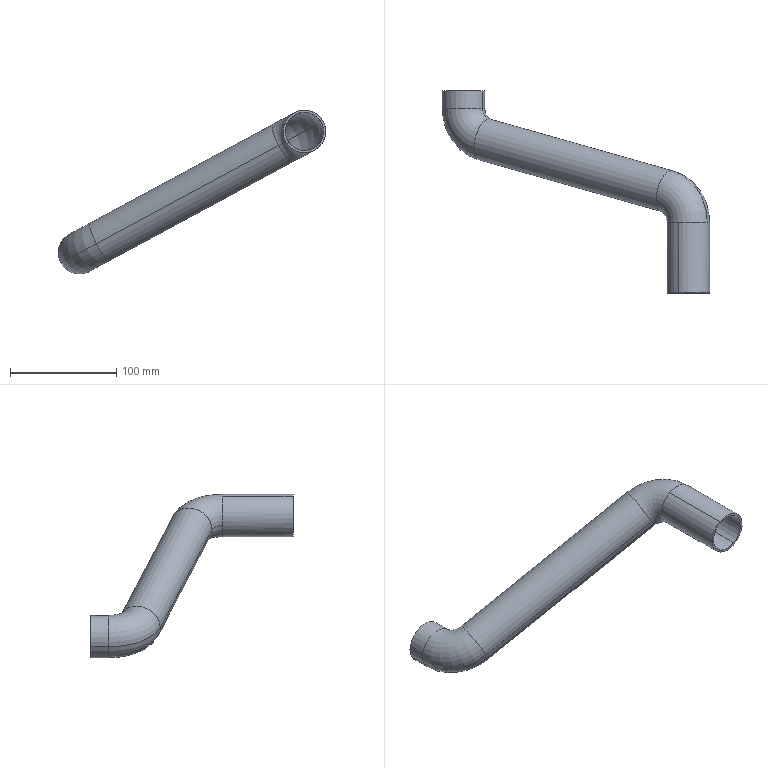Component | SolidWorks | SeedTube-1 | 1 solid | 22 faces | box 251.28 x 190 x 153.85 mm | volume 86728 mm3 | cylinder 12 | torus 8 | plane 2 | commonest cylinder face diameters 36 x6 40 x6
build123d program:
from build123d import *

# Parameters (mm, degrees)
SWEEP1_PROFILE_R = 20
SHELL1_T         = -2


with BuildPart() as part:
    # Sweep1: sweep along a curve in space
    with BuildLine() as sweep1_path:
        Line((0, 0, 0), (0, 66.577, 0))
        ThreePointArc((22.724, 95.681, 0), (6.354, 85.039, 0), (0, 66.577, 0))
        Line((22.724, 95.681, 0), (217.276, 144.319, 0))
        ThreePointArc((240, 173.423, 0), (233.646, 154.961, 0), (217.276, 144.319, 0))
        Line((240, 173.423, 0), (240, 190, 0))
    # Sweep1 profile (on start of the path) → Sweep1 (sweep)
    with BuildSketch(Plane.ZX):
        Circle(SWEEP1_PROFILE_R)
    sweep(path=sweep1_path.line)

    # Shell1
    shell1_openings = [part.faces().sort_by_distance(p)[0] for p in [
        (240, 190, 0),
        (0, 0, 0),
    ]]
    offset(amount=SHELL1_T, openings=shell1_openings, kind=Kind.INTERSECTION)


solid = part.part

# Placed as in the assembly
solid = solid.moved(Location((205.776, 72.5, -252.184), (180, 28.319, 180)))
STEP:
#1=COLOUR_RGB('',0.7922,0.8196,0.9333);
#2=FILL_AREA_STYLE_COLOUR('',#1);
#3=FILL_AREA_STYLE('',(#2));
#4=SURFACE_STYLE_FILL_AREA(#3);
#5=SURFACE_SIDE_STYLE('',(#4));
#6=SURFACE_STYLE_USAGE(.BOTH.,#5);
#7=PRESENTATION_STYLE_ASSIGNMENT((#6));
#8=CARTESIAN_POINT('',(0.7223,9.224,-13.905));
#9=VERTEX_POINT('',#8);
#10=CARTESIAN_POINT('',(0.4197,7.849,-14.068));
#11=VERTEX_POINT('',#10);
#12=CARTESIAN_POINT('',(0.571,8.536,-13.986));
#13=DIRECTION('',(0.854,-0.2425,0.4602));
#14=DIRECTION('',(0.2135,0.9701,0.1151));
#15=AXIS2_PLACEMENT_3D('',#12,#13,#14);
#16=CIRCLE('',#15,0.7087);
#17=EDGE_CURVE('',#9,#11,#16,.T.);
#18=ORIENTED_EDGE('',*,*,#17,.T.);
#19=CARTESIAN_POINT('',(-0.8404,9.682,-14.747));
#20=VERTEX_POINT('',#19);
#21=CARTESIAN_POINT('',(0.8232,9.682,-13.851));
#22=DIRECTION('',(0.4744,0.,-0.8803));
#23=DIRECTION('',(-0.8803,0.,-0.4744));
#24=AXIS2_PLACEMENT_3D('',#21,#22,#23);
#25=CIRCLE('',#24,1.89);
#26=EDGE_CURVE('',#11,#20,#25,.T.);
#27=ORIENTED_EDGE('',*,*,#26,.T.);
#28=CARTESIAN_POINT('',(0.4073,9.682,-14.075));
#29=VERTEX_POINT('',#28);
#30=CARTESIAN_POINT('',(-0.2165,9.682,-14.411));
#31=DIRECTION('',(0.,-1.,0.));
#32=DIRECTION('',(-0.4744,0.,0.8803));
#33=AXIS2_PLACEMENT_3D('',#30,#31,#32);
#34=CIRCLE('',#33,0.7087);
#35=EDGE_CURVE('',#29,#20,#34,.T.);
#36=ORIENTED_EDGE('',*,*,#35,.F.);
#37=CARTESIAN_POINT('',(0.8232,9.682,-13.851));
#38=DIRECTION('',(0.4744,0.,-0.8803));
#39=DIRECTION('',(-0.8803,0.,-0.4744));
#40=AXIS2_PLACEMENT_3D('',#37,#38,#39);
#41=CIRCLE('',#40,0.4724);
#42=EDGE_CURVE('',#9,#29,#41,.T.);
#43=ORIENTED_EDGE('',*,*,#42,.F.);
#44=EDGE_LOOP('',(#18,#27,#36,#43));
#45=FACE_OUTER_BOUND('',#44,.T.);
#46=CARTESIAN_POINT('',(0.8232,9.682,-13.851));
#47=DIRECTION('',(0.4744,0.,-0.8803));
#48=DIRECTION('',(-0.8803,0.,-0.4744));
#49=AXIS2_PLACEMENT_3D('',#46,#47,#48);
#50=TOROIDAL_SURFACE('',#49,1.181,0.7087);
#51=ADVANCED_FACE('',(#45),#50,.F.);
#52=CARTESIAN_POINT('',(8.438,5.475,-10.552));
#53=VERTEX_POINT('',#52);
#54=CARTESIAN_POINT('',(8.725,5.475,-9.592));
#55=VERTEX_POINT('',#54);
#56=CARTESIAN_POINT('',(8.101,5.475,-9.928));
#57=DIRECTION('',(0.,-1.,0.));
#58=DIRECTION('',(0.4744,0.,-0.8803));
#59=AXIS2_PLACEMENT_3D('',#56,#57,#58);
#60=CIRCLE('',#59,0.7087);
#61=EDGE_CURVE('',#53,#55,#60,.T.);
#62=ORIENTED_EDGE('',*,*,#61,.T.);
#63=CARTESIAN_POINT('',(7.465,7.309,-10.271));
#64=VERTEX_POINT('',#63);
#65=CARTESIAN_POINT('',(7.062,5.475,-10.489));
#66=DIRECTION('',(-0.4744,0.,0.8803));
#67=DIRECTION('',(0.8803,0.,0.4744));
#68=AXIS2_PLACEMENT_3D('',#65,#66,#67);
#69=CIRCLE('',#68,1.89);
#70=EDGE_CURVE('',#55,#64,#69,.T.);
#71=ORIENTED_EDGE('',*,*,#70,.T.);
#72=CARTESIAN_POINT('',(7.163,5.934,-10.434));
#73=VERTEX_POINT('',#72);
#74=CARTESIAN_POINT('',(7.314,6.621,-10.353));
#75=DIRECTION('',(0.854,-0.2425,0.4602));
#76=DIRECTION('',(-0.2135,-0.9701,-0.1151));
#77=AXIS2_PLACEMENT_3D('',#74,#75,#76);
#78=CIRCLE('',#77,0.7087);
#79=EDGE_CURVE('',#73,#64,#78,.T.);
#80=ORIENTED_EDGE('',*,*,#79,.F.);
#81=CARTESIAN_POINT('',(7.478,5.475,-10.265));
#82=VERTEX_POINT('',#81);
#83=CARTESIAN_POINT('',(7.062,5.475,-10.489));
#84=DIRECTION('',(-0.4744,0.,0.8803));
#85=DIRECTION('',(0.8803,0.,0.4744));
#86=AXIS2_PLACEMENT_3D('',#83,#84,#85);
#87=CIRCLE('',#86,0.4724);
#88=EDGE_CURVE('',#82,#73,#87,.T.);
#89=ORIENTED_EDGE('',*,*,#88,.F.);
#90=CARTESIAN_POINT('',(8.101,5.475,-9.928));
#91=DIRECTION('',(0.,-1.,0.));
#92=DIRECTION('',(0.4744,0.,-0.8803));
#93=AXIS2_PLACEMENT_3D('',#90,#91,#92);
#94=CIRCLE('',#93,0.7087);
#95=EDGE_CURVE('',#82,#53,#94,.T.);
#96=ORIENTED_EDGE('',*,*,#95,.T.);
#97=EDGE_LOOP('',(#62,#71,#80,#89,#96));
#98=FACE_OUTER_BOUND('',#97,.T.);
#99=CARTESIAN_POINT('',(7.062,5.475,-10.489));
#100=DIRECTION('',(-0.4744,0.,0.8803));
#101=DIRECTION('',(0.8803,0.,0.4744));
#102=AXIS2_PLACEMENT_3D('',#99,#100,#101);
#103=TOROIDAL_SURFACE('',#102,1.181,0.7087);
#104=ADVANCED_FACE('',(#98),#103,.F.);
#105=CARTESIAN_POINT('',(0.4029,7.772,-14.077));
#106=VERTEX_POINT('',#105);
#107=CARTESIAN_POINT('',(0.7392,9.3,-13.896));
#108=VERTEX_POINT('',#107);
#109=CARTESIAN_POINT('',(0.571,8.536,-13.986));
#110=DIRECTION('',(0.854,-0.2425,0.4602));
#111=DIRECTION('',(-0.4744,0.,0.8803));
#112=AXIS2_PLACEMENT_3D('',#109,#110,#111);
#113=CIRCLE('',#112,0.7874);
#114=EDGE_CURVE('',#106,#108,#113,.T.);
#115=ORIENTED_EDGE('',*,*,#114,.F.);
#116=CARTESIAN_POINT('',(-0.9097,9.682,-14.784));
#117=VERTEX_POINT('',#116);
#118=CARTESIAN_POINT('',(0.8232,9.682,-13.851));
#119=DIRECTION('',(0.4744,0.,-0.8803));
#120=DIRECTION('',(-0.8803,0.,-0.4744));
#121=AXIS2_PLACEMENT_3D('',#118,#119,#120);
#122=CIRCLE('',#121,1.969);
#123=EDGE_CURVE('',#106,#117,#122,.T.);
#124=ORIENTED_EDGE('',*,*,#123,.T.);
#125=CARTESIAN_POINT('',(0.4766,9.682,-14.037));
#126=VERTEX_POINT('',#125);
#127=CARTESIAN_POINT('',(-0.2165,9.682,-14.411));
#128=DIRECTION('',(-0.,-1.,0.));
#129=DIRECTION('',(-0.4744,0.,0.8803));
#130=AXIS2_PLACEMENT_3D('',#127,#128,#129);
#131=CIRCLE('',#130,0.7874);
#132=EDGE_CURVE('',#117,#126,#131,.T.);
#133=ORIENTED_EDGE('',*,*,#132,.T.);
#134=CARTESIAN_POINT('',(0.8232,9.682,-13.851));
#135=DIRECTION('',(0.4744,0.,-0.8803));
#136=DIRECTION('',(-0.8803,0.,-0.4744));
#137=AXIS2_PLACEMENT_3D('',#134,#135,#136);
#138=CIRCLE('',#137,0.3937);
#139=EDGE_CURVE('',#108,#126,#138,.T.);
#140=ORIENTED_EDGE('',*,*,#139,.F.);
#141=EDGE_LOOP('',(#115,#124,#133,#140));
#142=FACE_OUTER_BOUND('',#141,.T.);
#143=CARTESIAN_POINT('',(0.8232,9.682,-13.851));
#144=DIRECTION('',(0.4744,0.,-0.8803));
#145=DIRECTION('',(-0.8803,0.,-0.4744));
#146=AXIS2_PLACEMENT_3D('',#143,#144,#145);
#147=TOROIDAL_SURFACE('',#146,1.181,0.7874);
#148=ADVANCED_FACE('',(#142),#147,.T.);
#149=CARTESIAN_POINT('',(8.795,5.475,-9.555));
#150=VERTEX_POINT('',#149);
#151=CARTESIAN_POINT('',(7.728,5.475,-9.235));
#152=VERTEX_POINT('',#151);
#153=CARTESIAN_POINT('',(8.101,5.475,-9.928));
#154=DIRECTION('',(-0.,-1.,0.));
#155=DIRECTION('',(-0.4744,0.,0.8803));
#156=AXIS2_PLACEMENT_3D('',#153,#154,#155);
#157=CIRCLE('',#156,0.7874);
#158=EDGE_CURVE('',#150,#152,#157,.T.);
#159=ORIENTED_EDGE('',*,*,#158,.F.);
#160=CARTESIAN_POINT('',(7.482,7.385,-10.262));
#161=VERTEX_POINT('',#160);
#162=CARTESIAN_POINT('',(7.062,5.475,-10.489));
#163=DIRECTION('',(-0.4744,0.,0.8803));
#164=DIRECTION('',(0.8803,0.,0.4744));
#165=AXIS2_PLACEMENT_3D('',#162,#163,#164);
#166=CIRCLE('',#165,1.969);
#167=EDGE_CURVE('',#150,#161,#166,.T.);
#168=ORIENTED_EDGE('',*,*,#167,.T.);
#169=CARTESIAN_POINT('',(7.146,5.857,-10.443));
#170=VERTEX_POINT('',#169);
#171=CARTESIAN_POINT('',(7.314,6.621,-10.353));
#172=DIRECTION('',(0.854,-0.2425,0.4602));
#173=DIRECTION('',(-0.4744,0.,0.8803));
#174=AXIS2_PLACEMENT_3D('',#171,#172,#173);
#175=CIRCLE('',#174,0.7874);
#176=EDGE_CURVE('',#161,#170,#175,.T.);
#177=ORIENTED_EDGE('',*,*,#176,.T.);
#178=CARTESIAN_POINT('',(7.408,5.475,-10.302));
#179=VERTEX_POINT('',#178);
#180=CARTESIAN_POINT('',(7.062,5.475,-10.489));
#181=DIRECTION('',(-0.4744,0.,0.8803));
#182=DIRECTION('',(0.8803,0.,0.4744));
#183=AXIS2_PLACEMENT_3D('',#180,#181,#182);
#184=CIRCLE('',#183,0.3937);
#185=EDGE_CURVE('',#179,#170,#184,.T.);
#186=ORIENTED_EDGE('',*,*,#185,.F.);
#187=CARTESIAN_POINT('',(8.101,5.475,-9.928));
#188=DIRECTION('',(-0.,-1.,0.));
#189=DIRECTION('',(-0.4744,0.,0.8803));
#190=AXIS2_PLACEMENT_3D('',#187,#188,#189);
#191=CIRCLE('',#190,0.7874);
#192=EDGE_CURVE('',#152,#179,#191,.T.);
#193=ORIENTED_EDGE('',*,*,#192,.F.);
#194=EDGE_LOOP('',(#159,#168,#177,#186,#193));
#195=FACE_OUTER_BOUND('',#194,.T.);
#196=CARTESIAN_POINT('',(7.062,5.475,-10.489));
#197=DIRECTION('',(-0.4744,0.,0.8803));
#198=DIRECTION('',(0.8803,0.,0.4744));
#199=AXIS2_PLACEMENT_3D('',#196,#197,#198);
#200=TOROIDAL_SURFACE('',#199,1.181,0.7874);
#201=ADVANCED_FACE('',(#195),#200,.T.);
#202=ORIENTED_EDGE('',*,*,#35,.T.);
#203=CARTESIAN_POINT('',(-0.8404,10.335,-14.747));
#204=VERTEX_POINT('',#203);
#205=CARTESIAN_POINT('',(-0.8404,9.682,-14.747));
#206=DIRECTION('',(0.,1.,0.));
#207=VECTOR('',#206,39.37);
#208=LINE('',#205,#207);
#209=EDGE_CURVE('',#20,#204,#208,.T.);
#210=ORIENTED_EDGE('',*,*,#209,.T.);
#211=CARTESIAN_POINT('',(0.4073,10.335,-14.075));
#212=VERTEX_POINT('',#211);
#213=CARTESIAN_POINT('',(-0.2165,10.335,-14.411));
#214=DIRECTION('',(-0.,-1.,0.));
#215=DIRECTION('',(-0.4744,0.,0.8803));
#216=AXIS2_PLACEMENT_3D('',#213,#214,#215);
#217=CIRCLE('',#216,0.7087);
#218=EDGE_CURVE('',#212,#204,#217,.T.);
#219=ORIENTED_EDGE('',*,*,#218,.F.);
#220=CARTESIAN_POINT('',(0.4073,9.682,-14.075));
#221=DIRECTION('',(0.,1.,0.));
#222=VECTOR('',#221,39.37);
#223=LINE('',#220,#222);
#224=EDGE_CURVE('',#29,#212,#223,.T.);
#225=ORIENTED_EDGE('',*,*,#224,.F.);
#226=EDGE_LOOP('',(#202,#210,#219,#225));
#227=FACE_OUTER_BOUND('',#226,.T.);
#228=CARTESIAN_POINT('',(-0.2165,9.682,-14.411));
#229=DIRECTION('',(0.,1.,0.));
#230=DIRECTION('',(0.8803,-0.,0.4744));
#231=AXIS2_PLACEMENT_3D('',#228,#229,#230);
#232=CYLINDRICAL_SURFACE('',#231,0.7087);
#233=ADVANCED_FACE('',(#227),#232,.F.);
#234=CARTESIAN_POINT('',(7.314,6.621,-10.353));
#235=DIRECTION('',(0.854,-0.2425,0.4602));
#236=DIRECTION('',(-0.2135,-0.9701,-0.1151));
#237=AXIS2_PLACEMENT_3D('',#234,#235,#236);
#238=CIRCLE('',#237,0.7087);
#239=EDGE_CURVE('',#64,#73,#238,.T.);
#240=ORIENTED_EDGE('',*,*,#239,.T.);
#241=CARTESIAN_POINT('',(7.163,5.934,-10.434));
#242=DIRECTION('',(-0.854,0.2425,-0.4602));
#243=VECTOR('',#242,39.37);
#244=LINE('',#241,#243);
#245=EDGE_CURVE('',#73,#11,#244,.T.);
#246=ORIENTED_EDGE('',*,*,#245,.T.);
#247=ORIENTED_EDGE('',*,*,#17,.F.);
#248=CARTESIAN_POINT('',(7.465,7.309,-10.271));
#249=DIRECTION('',(-0.854,0.2425,-0.4602));
#250=VECTOR('',#249,39.37);
#251=LINE('',#248,#250);
#252=EDGE_CURVE('',#64,#9,#251,.T.);
#253=ORIENTED_EDGE('',*,*,#252,.F.);
#254=EDGE_LOOP('',(#240,#246,#247,#253));
#255=FACE_OUTER_BOUND('',#254,.T.);
#256=CARTESIAN_POINT('',(7.314,6.621,-10.353));
#257=DIRECTION('',(-0.854,0.2425,-0.4602));
#258=DIRECTION('',(0.2135,0.9701,0.1151));
#259=AXIS2_PLACEMENT_3D('',#256,#257,#258);
#260=CYLINDRICAL_SURFACE('',#259,0.7087);
#261=ADVANCED_FACE('',(#255),#260,.F.);
#262=CARTESIAN_POINT('',(8.438,2.854,-10.552));
#263=VERTEX_POINT('',#262);
#264=CARTESIAN_POINT('',(7.765,2.854,-9.305));
#265=VERTEX_POINT('',#264);
#266=CARTESIAN_POINT('',(8.101,2.854,-9.928));
#267=DIRECTION('',(-0.,-1.,0.));
#268=DIRECTION('',(-0.4744,0.,0.8803));
#269=AXIS2_PLACEMENT_3D('',#266,#267,#268);
#270=CIRCLE('',#269,0.7087);
#271=EDGE_CURVE('',#263,#265,#270,.T.);
#272=ORIENTED_EDGE('',*,*,#271,.T.);
#273=CARTESIAN_POINT('',(7.765,5.475,-9.305));
#274=VERTEX_POINT('',#273);
#275=CARTESIAN_POINT('',(7.765,2.854,-9.305));
#276=DIRECTION('',(0.,1.,0.));
#277=VECTOR('',#276,39.37);
#278=LINE('',#275,#277);
#279=EDGE_CURVE('',#265,#274,#278,.T.);
#280=ORIENTED_EDGE('',*,*,#279,.T.);
#281=CARTESIAN_POINT('',(8.101,5.475,-9.928));
#282=DIRECTION('',(0.,-1.,0.));
#283=DIRECTION('',(0.4744,0.,-0.8803));
#284=AXIS2_PLACEMENT_3D('',#281,#282,#283);
#285=CIRCLE('',#284,0.7087);
#286=EDGE_CURVE('',#55,#274,#285,.T.);
#287=ORIENTED_EDGE('',*,*,#286,.F.);
#288=ORIENTED_EDGE('',*,*,#61,.F.);
#289=CARTESIAN_POINT('',(8.438,2.854,-10.552));
#290=DIRECTION('',(0.,1.,0.));
#291=VECTOR('',#290,39.37);
#292=LINE('',#289,#291);
#293=EDGE_CURVE('',#263,#53,#292,.T.);
#294=ORIENTED_EDGE('',*,*,#293,.F.);
#295=EDGE_LOOP('',(#272,#280,#287,#288,#294));
#296=FACE_OUTER_BOUND('',#295,.T.);
#297=CARTESIAN_POINT('',(8.101,2.854,-9.928));
#298=DIRECTION('',(0.,1.,0.));
#299=DIRECTION('',(0.4744,0.,-0.8803));
#300=AXIS2_PLACEMENT_3D('',#297,#298,#299);
#301=CYLINDRICAL_SURFACE('',#300,0.7087);
#302=ADVANCED_FACE('',(#296),#301,.F.);
#303=ORIENTED_EDGE('',*,*,#132,.F.);
#304=CARTESIAN_POINT('',(-0.9097,10.335,-14.784));
#305=VERTEX_POINT('',#304);
#306=CARTESIAN_POINT('',(-0.9097,9.682,-14.784));
#307=DIRECTION('',(0.,1.,0.));
#308=VECTOR('',#307,39.37);
#309=LINE('',#306,#308);
#310=EDGE_CURVE('',#117,#305,#309,.T.);
#311=ORIENTED_EDGE('',*,*,#310,.T.);
#312=CARTESIAN_POINT('',(0.4766,10.335,-14.037));
#313=VERTEX_POINT('',#312);
#314=CARTESIAN_POINT('',(-0.2165,10.335,-14.411));
#315=DIRECTION('',(-0.,-1.,0.));
#316=DIRECTION('',(-0.4744,0.,0.8803));
#317=AXIS2_PLACEMENT_3D('',#314,#315,#316);
#318=CIRCLE('',#317,0.7874);
#319=EDGE_CURVE('',#305,#313,#318,.T.);
#320=ORIENTED_EDGE('',*,*,#319,.T.);
#321=CARTESIAN_POINT('',(0.4766,9.682,-14.037));
#322=DIRECTION('',(0.,1.,0.));
#323=VECTOR('',#322,39.37);
#324=LINE('',#321,#323);
#325=EDGE_CURVE('',#126,#313,#324,.T.);
#326=ORIENTED_EDGE('',*,*,#325,.F.);
#327=EDGE_LOOP('',(#303,#311,#320,#326));
#328=FACE_OUTER_BOUND('',#327,.T.);
#329=CARTESIAN_POINT('',(-0.2165,9.682,-14.411));
#330=DIRECTION('',(0.,1.,0.));
#331=DIRECTION('',(0.8803,-0.,0.4744));
#332=AXIS2_PLACEMENT_3D('',#329,#330,#331);
#333=CYLINDRICAL_SURFACE('',#332,0.7874);
#334=ADVANCED_FACE('',(#328),#333,.T.);
#335=CARTESIAN_POINT('',(7.314,6.621,-10.353));
#336=DIRECTION('',(0.854,-0.2425,0.4602));
#337=DIRECTION('',(-0.4744,0.,0.8803));
#338=AXIS2_PLACEMENT_3D('',#335,#336,#337);
#339=CIRCLE('',#338,0.7874);
#340=EDGE_CURVE('',#170,#161,#339,.T.);
#341=ORIENTED_EDGE('',*,*,#340,.F.);
#342=CARTESIAN_POINT('',(7.146,5.857,-10.443));
#343=DIRECTION('',(-0.854,0.2425,-0.4602));
#344=VECTOR('',#343,39.37);
#345=LINE('',#342,#344);
#346=EDGE_CURVE('',#170,#106,#345,.T.);
#347=ORIENTED_EDGE('',*,*,#346,.T.);
#348=ORIENTED_EDGE('',*,*,#114,.T.);
#349=CARTESIAN_POINT('',(7.482,7.385,-10.262));
#350=DIRECTION('',(-0.854,0.2425,-0.4602));
#351=VECTOR('',#350,39.37);
#352=LINE('',#349,#351);
#353=EDGE_CURVE('',#161,#108,#352,.T.);
#354=ORIENTED_EDGE('',*,*,#353,.F.);
#355=EDGE_LOOP('',(#341,#347,#348,#354));
#356=FACE_OUTER_BOUND('',#355,.T.);
#357=CARTESIAN_POINT('',(7.314,6.621,-10.353));
#358=DIRECTION('',(-0.854,0.2425,-0.4602));
#359=DIRECTION('',(0.2135,0.9701,0.1151));
#360=AXIS2_PLACEMENT_3D('',#357,#358,#359);
#361=CYLINDRICAL_SURFACE('',#360,0.7874);
#362=ADVANCED_FACE('',(#356),#361,.T.);
#363=CARTESIAN_POINT('',(7.728,2.854,-9.235));
#364=VERTEX_POINT('',#363);
#365=CARTESIAN_POINT('',(8.475,2.854,-10.622));
#366=VERTEX_POINT('',#365);
#367=CARTESIAN_POINT('',(8.101,2.854,-9.928));
#368=DIRECTION('',(-0.,-1.,0.));
#369=DIRECTION('',(-0.4744,0.,0.8803));
#370=AXIS2_PLACEMENT_3D('',#367,#368,#369);
#371=CIRCLE('',#370,0.7874);
#372=EDGE_CURVE('',#364,#366,#371,.T.);
#373=ORIENTED_EDGE('',*,*,#372,.F.);
#374=CARTESIAN_POINT('',(7.728,2.854,-9.235));
#375=DIRECTION('',(0.,1.,0.));
#376=VECTOR('',#375,39.37);
#377=LINE('',#374,#376);
#378=EDGE_CURVE('',#364,#152,#377,.T.);
#379=ORIENTED_EDGE('',*,*,#378,.T.);
#380=ORIENTED_EDGE('',*,*,#192,.T.);
#381=CARTESIAN_POINT('',(8.475,5.475,-10.622));
#382=VERTEX_POINT('',#381);
#383=CARTESIAN_POINT('',(8.101,5.475,-9.928));
#384=DIRECTION('',(-0.,-1.,0.));
#385=DIRECTION('',(-0.4744,0.,0.8803));
#386=AXIS2_PLACEMENT_3D('',#383,#384,#385);
#387=CIRCLE('',#386,0.7874);
#388=EDGE_CURVE('',#179,#382,#387,.T.);
#389=ORIENTED_EDGE('',*,*,#388,.T.);
#390=CARTESIAN_POINT('',(8.475,2.854,-10.622));
#391=DIRECTION('',(0.,1.,0.));
#392=VECTOR('',#391,39.37);
#393=LINE('',#390,#392);
#394=EDGE_CURVE('',#366,#382,#393,.T.);
#395=ORIENTED_EDGE('',*,*,#394,.F.);
#396=EDGE_LOOP('',(#373,#379,#380,#389,#395));
#397=FACE_OUTER_BOUND('',#396,.T.);
#398=CARTESIAN_POINT('',(8.101,2.854,-9.928));
#399=DIRECTION('',(0.,1.,0.));
#400=DIRECTION('',(0.4744,0.,-0.8803));
#401=AXIS2_PLACEMENT_3D('',#398,#399,#400);
#402=CYLINDRICAL_SURFACE('',#401,0.7874);
#403=ADVANCED_FACE('',(#397),#402,.T.);
#404=ORIENTED_EDGE('',*,*,#310,.F.);
#405=CARTESIAN_POINT('',(-0.2165,9.682,-14.411));
#406=DIRECTION('',(-0.,-1.,0.));
#407=DIRECTION('',(-0.4744,0.,0.8803));
#408=AXIS2_PLACEMENT_3D('',#405,#406,#407);
#409=CIRCLE('',#408,0.7874);
#410=EDGE_CURVE('',#126,#117,#409,.T.);
#411=ORIENTED_EDGE('',*,*,#410,.F.);
#412=ORIENTED_EDGE('',*,*,#325,.T.);
#413=CARTESIAN_POINT('',(-0.2165,10.335,-14.411));
#414=DIRECTION('',(-0.,-1.,0.));
#415=DIRECTION('',(-0.4744,0.,0.8803));
#416=AXIS2_PLACEMENT_3D('',#413,#414,#415);
#417=CIRCLE('',#416,0.7874);
#418=EDGE_CURVE('',#313,#305,#417,.T.);
#419=ORIENTED_EDGE('',*,*,#418,.T.);
#420=EDGE_LOOP('',(#404,#411,#412,#419));
#421=FACE_OUTER_BOUND('',#420,.T.);
#422=CARTESIAN_POINT('',(-0.2165,9.682,-14.411));
#423=DIRECTION('',(0.,1.,0.));
#424=DIRECTION('',(0.8803,-0.,0.4744));
#425=AXIS2_PLACEMENT_3D('',#422,#423,#424);
#426=CYLINDRICAL_SURFACE('',#425,0.7874);
#427=ADVANCED_FACE('',(#421),#426,.T.);
#428=ORIENTED_EDGE('',*,*,#123,.F.);
#429=CARTESIAN_POINT('',(0.571,8.536,-13.986));
#430=DIRECTION('',(0.854,-0.2425,0.4602));
#431=DIRECTION('',(-0.4744,0.,0.8803));
#432=AXIS2_PLACEMENT_3D('',#429,#430,#431);
#433=CIRCLE('',#432,0.7874);
#434=EDGE_CURVE('',#108,#106,#433,.T.);
#435=ORIENTED_EDGE('',*,*,#434,.F.);
#436=ORIENTED_EDGE('',*,*,#139,.T.);
#437=ORIENTED_EDGE('',*,*,#410,.T.);
#438=EDGE_LOOP('',(#428,#435,#436,#437));
#439=FACE_OUTER_BOUND('',#438,.T.);
#440=CARTESIAN_POINT('',(0.8232,9.682,-13.851));
#441=DIRECTION('',(0.4744,0.,-0.8803));
#442=DIRECTION('',(-0.8803,0.,-0.4744));
#443=AXIS2_PLACEMENT_3D('',#440,#441,#442);
#444=TOROIDAL_SURFACE('',#443,1.181,0.7874);
#445=ADVANCED_FACE('',(#439),#444,.T.);
#446=ORIENTED_EDGE('',*,*,#346,.F.);
#447=ORIENTED_EDGE('',*,*,#176,.F.);
#448=ORIENTED_EDGE('',*,*,#353,.T.);
#449=ORIENTED_EDGE('',*,*,#434,.T.);
#450=EDGE_LOOP('',(#446,#447,#448,#449));
#451=FACE_OUTER_BOUND('',#450,.T.);
#452=CARTESIAN_POINT('',(7.314,6.621,-10.353));
#453=DIRECTION('',(-0.854,0.2425,-0.4602));
#454=DIRECTION('',(0.2135,0.9701,0.1151));
#455=AXIS2_PLACEMENT_3D('',#452,#453,#454);
#456=CYLINDRICAL_SURFACE('',#455,0.7874);
#457=ADVANCED_FACE('',(#451),#456,.T.);
#458=ORIENTED_EDGE('',*,*,#167,.F.);
#459=CARTESIAN_POINT('',(8.101,5.475,-9.928));
#460=DIRECTION('',(-0.,-1.,0.));
#461=DIRECTION('',(-0.4744,0.,0.8803));
#462=AXIS2_PLACEMENT_3D('',#459,#460,#461);
#463=CIRCLE('',#462,0.7874);
#464=EDGE_CURVE('',#382,#150,#463,.T.);
#465=ORIENTED_EDGE('',*,*,#464,.F.);
#466=ORIENTED_EDGE('',*,*,#388,.F.);
#467=ORIENTED_EDGE('',*,*,#185,.T.);
#468=ORIENTED_EDGE('',*,*,#340,.T.);
#469=EDGE_LOOP('',(#458,#465,#466,#467,#468));
#470=FACE_OUTER_BOUND('',#469,.T.);
#471=CARTESIAN_POINT('',(7.062,5.475,-10.489));
#472=DIRECTION('',(-0.4744,0.,0.8803));
#473=DIRECTION('',(0.8803,0.,0.4744));
#474=AXIS2_PLACEMENT_3D('',#471,#472,#473);
#475=TOROIDAL_SURFACE('',#474,1.181,0.7874);
#476=ADVANCED_FACE('',(#470),#475,.T.);
#477=ORIENTED_EDGE('',*,*,#378,.F.);
#478=CARTESIAN_POINT('',(8.101,2.854,-9.928));
#479=DIRECTION('',(-0.,-1.,0.));
#480=DIRECTION('',(-0.4744,0.,0.8803));
#481=AXIS2_PLACEMENT_3D('',#478,#479,#480);
#482=CIRCLE('',#481,0.7874);
#483=EDGE_CURVE('',#366,#364,#482,.T.);
#484=ORIENTED_EDGE('',*,*,#483,.F.);
#485=ORIENTED_EDGE('',*,*,#394,.T.);
#486=ORIENTED_EDGE('',*,*,#464,.T.);
#487=ORIENTED_EDGE('',*,*,#158,.T.);
#488=EDGE_LOOP('',(#477,#484,#485,#486,#487));
#489=FACE_OUTER_BOUND('',#488,.T.);
#490=CARTESIAN_POINT('',(8.101,2.854,-9.928));
#491=DIRECTION('',(0.,1.,0.));
#492=DIRECTION('',(0.4744,0.,-0.8803));
#493=AXIS2_PLACEMENT_3D('',#490,#491,#492);
#494=CYLINDRICAL_SURFACE('',#493,0.7874);
#495=ADVANCED_FACE('',(#489),#494,.T.);
#496=ORIENTED_EDGE('',*,*,#218,.T.);
#497=CARTESIAN_POINT('',(-0.2165,10.335,-14.411));
#498=DIRECTION('',(-0.,-1.,0.));
#499=DIRECTION('',(-0.4744,0.,0.8803));
#500=AXIS2_PLACEMENT_3D('',#497,#498,#499);
#501=CIRCLE('',#500,0.7087);
#502=EDGE_CURVE('',#204,#212,#501,.T.);
#503=ORIENTED_EDGE('',*,*,#502,.T.);
#504=EDGE_LOOP('',(#496,#503));
#505=FACE_BOUND('',#504,.T.);
#506=ORIENTED_EDGE('',*,*,#418,.F.);
#507=ORIENTED_EDGE('',*,*,#319,.F.);
#508=EDGE_LOOP('',(#506,#507));
#509=FACE_OUTER_BOUND('',#508,.T.);
#510=CARTESIAN_POINT('',(-0.2165,10.335,-14.411));
#511=DIRECTION('',(-0.,-1.,0.));
#512=DIRECTION('',(-0.4744,0.,0.8803));
#513=AXIS2_PLACEMENT_3D('',#510,#511,#512);
#514=PLANE('',#513);
#515=ADVANCED_FACE('',(#505,#509),#514,.F.);
#516=ORIENTED_EDGE('',*,*,#271,.F.);
#517=CARTESIAN_POINT('',(8.101,2.854,-9.928));
#518=DIRECTION('',(-0.,-1.,0.));
#519=DIRECTION('',(-0.4744,0.,0.8803));
#520=AXIS2_PLACEMENT_3D('',#517,#518,#519);
#521=CIRCLE('',#520,0.7087);
#522=EDGE_CURVE('',#265,#263,#521,.T.);
#523=ORIENTED_EDGE('',*,*,#522,.F.);
#524=EDGE_LOOP('',(#516,#523));
#525=FACE_BOUND('',#524,.T.);
#526=ORIENTED_EDGE('',*,*,#483,.T.);
#527=ORIENTED_EDGE('',*,*,#372,.T.);
#528=EDGE_LOOP('',(#526,#527));
#529=FACE_OUTER_BOUND('',#528,.T.);
#530=CARTESIAN_POINT('',(8.101,2.854,-9.928));
#531=DIRECTION('',(-0.,-1.,0.));
#532=DIRECTION('',(-0.4744,0.,0.8803));
#533=AXIS2_PLACEMENT_3D('',#530,#531,#532);
#534=PLANE('',#533);
#535=ADVANCED_FACE('',(#525,#529),#534,.T.);
#536=ORIENTED_EDGE('',*,*,#209,.F.);
#537=CARTESIAN_POINT('',(-0.2165,9.682,-14.411));
#538=DIRECTION('',(0.,-1.,0.));
#539=DIRECTION('',(-0.4744,0.,0.8803));
#540=AXIS2_PLACEMENT_3D('',#537,#538,#539);
#541=CIRCLE('',#540,0.7087);
#542=EDGE_CURVE('',#20,#29,#541,.T.);
#543=ORIENTED_EDGE('',*,*,#542,.T.);
#544=ORIENTED_EDGE('',*,*,#224,.T.);
#545=ORIENTED_EDGE('',*,*,#502,.F.);
#546=EDGE_LOOP('',(#536,#543,#544,#545));
#547=FACE_OUTER_BOUND('',#546,.T.);
#548=CARTESIAN_POINT('',(-0.2165,9.682,-14.411));
#549=DIRECTION('',(0.,1.,0.));
#550=DIRECTION('',(0.8803,-0.,0.4744));
#551=AXIS2_PLACEMENT_3D('',#548,#549,#550);
#552=CYLINDRICAL_SURFACE('',#551,0.7087);
#553=ADVANCED_FACE('',(#547),#552,.F.);
#554=ORIENTED_EDGE('',*,*,#26,.F.);
#555=CARTESIAN_POINT('',(0.571,8.536,-13.986));
#556=DIRECTION('',(0.854,-0.2425,0.4602));
#557=DIRECTION('',(0.2135,0.9701,0.1151));
#558=AXIS2_PLACEMENT_3D('',#555,#556,#557);
#559=CIRCLE('',#558,0.7087);
#560=EDGE_CURVE('',#11,#9,#559,.T.);
#561=ORIENTED_EDGE('',*,*,#560,.T.);
#562=ORIENTED_EDGE('',*,*,#42,.T.);
#563=ORIENTED_EDGE('',*,*,#542,.F.);
#564=EDGE_LOOP('',(#554,#561,#562,#563));
#565=FACE_OUTER_BOUND('',#564,.T.);
#566=CARTESIAN_POINT('',(0.8232,9.682,-13.851));
#567=DIRECTION('',(0.4744,0.,-0.8803));
#568=DIRECTION('',(-0.8803,0.,-0.4744));
#569=AXIS2_PLACEMENT_3D('',#566,#567,#568);
#570=TOROIDAL_SURFACE('',#569,1.181,0.7087);
#571=ADVANCED_FACE('',(#565),#570,.F.);
#572=ORIENTED_EDGE('',*,*,#245,.F.);
#573=ORIENTED_EDGE('',*,*,#79,.T.);
#574=ORIENTED_EDGE('',*,*,#252,.T.);
#575=ORIENTED_EDGE('',*,*,#560,.F.);
#576=EDGE_LOOP('',(#572,#573,#574,#575));
#577=FACE_OUTER_BOUND('',#576,.T.);
#578=CARTESIAN_POINT('',(7.314,6.621,-10.353));
#579=DIRECTION('',(-0.854,0.2425,-0.4602));
#580=DIRECTION('',(0.2135,0.9701,0.1151));
#581=AXIS2_PLACEMENT_3D('',#578,#579,#580);
#582=CYLINDRICAL_SURFACE('',#581,0.7087);
#583=ADVANCED_FACE('',(#577),#582,.F.);
#584=ORIENTED_EDGE('',*,*,#70,.F.);
#585=ORIENTED_EDGE('',*,*,#286,.T.);
#586=CARTESIAN_POINT('',(8.101,5.475,-9.928));
#587=DIRECTION('',(0.,-1.,0.));
#588=DIRECTION('',(0.4744,0.,-0.8803));
#589=AXIS2_PLACEMENT_3D('',#586,#587,#588);
#590=CIRCLE('',#589,0.7087);
#591=EDGE_CURVE('',#274,#82,#590,.T.);
#592=ORIENTED_EDGE('',*,*,#591,.T.);
#593=ORIENTED_EDGE('',*,*,#88,.T.);
#594=ORIENTED_EDGE('',*,*,#239,.F.);
#595=EDGE_LOOP('',(#584,#585,#592,#593,#594));
#596=FACE_OUTER_BOUND('',#595,.T.);
#597=CARTESIAN_POINT('',(7.062,5.475,-10.489));
#598=DIRECTION('',(-0.4744,0.,0.8803));
#599=DIRECTION('',(0.8803,0.,0.4744));
#600=AXIS2_PLACEMENT_3D('',#597,#598,#599);
#601=TOROIDAL_SURFACE('',#600,1.181,0.7087);
#602=ADVANCED_FACE('',(#596),#601,.F.);
#603=ORIENTED_EDGE('',*,*,#279,.F.);
#604=ORIENTED_EDGE('',*,*,#522,.T.);
#605=ORIENTED_EDGE('',*,*,#293,.T.);
#606=ORIENTED_EDGE('',*,*,#95,.F.);
#607=ORIENTED_EDGE('',*,*,#591,.F.);
#608=EDGE_LOOP('',(#603,#604,#605,#606,#607));
#609=FACE_OUTER_BOUND('',#608,.T.);
#610=CARTESIAN_POINT('',(8.101,2.854,-9.928));
#611=DIRECTION('',(0.,1.,0.));
#612=DIRECTION('',(0.4744,0.,-0.8803));
#613=AXIS2_PLACEMENT_3D('',#610,#611,#612);
#614=CYLINDRICAL_SURFACE('',#613,0.7087);
#615=ADVANCED_FACE('',(#609),#614,.F.);
#616=CLOSED_SHELL('',(#51,#104,#148,#201,#233,#261,#302,#334,#362,#403,#427,#445,#457,#476,#495,#515,#535,#553,#571,#583,#602,#615));
#617=MANIFOLD_SOLID_BREP('',#616);
#618=STYLED_ITEM('',(#7),#617);
#619=(LENGTH_UNIT()NAMED_UNIT(*)SI_UNIT($,.METRE.));
#620=LENGTH_MEASURE_WITH_UNIT(LENGTH_MEASURE(0.0254),#619);
#621=DIMENSIONAL_EXPONENTS(1.,0.,0.,0.,0.,0.,0.);
#622=(CONVERSION_BASED_UNIT('',#620)LENGTH_UNIT()NAMED_UNIT(#621));
#623=UNCERTAINTY_MEASURE_WITH_UNIT(LENGTH_MEASURE(0.00001),#622,'','');
#624=(NAMED_UNIT(*)PLANE_ANGLE_UNIT()SI_UNIT($,.RADIAN.));
#625=(NAMED_UNIT(*)SI_UNIT($,.STERADIAN.)SOLID_ANGLE_UNIT());
#626=(GEOMETRIC_REPRESENTATION_CONTEXT(3)GLOBAL_UNCERTAINTY_ASSIGNED_CONTEXT((#623))GLOBAL_UNIT_ASSIGNED_CONTEXT((#622,#624,#625))REPRESENTATION_CONTEXT('',''));
#627=MECHANICAL_DESIGN_GEOMETRIC_PRESENTATION_REPRESENTATION('',(#618),#626);
#628=PRESENTATION_LAYER_ASSIGNMENT('','',(#618));
#629=CARTESIAN_POINT('',(0.,0.,0.));
#630=DIRECTION('',(0.,0.,1.));
#631=DIRECTION('',(1.,0.,0.));
#632=AXIS2_PLACEMENT_3D('',#629,#630,#631);
#633=(LENGTH_UNIT()NAMED_UNIT(*)SI_UNIT($,.METRE.));
#634=LENGTH_MEASURE_WITH_UNIT(LENGTH_MEASURE(0.0254),#633);
#635=DIMENSIONAL_EXPONENTS(1.,0.,0.,0.,0.,0.,0.);
#636=(CONVERSION_BASED_UNIT('',#634)LENGTH_UNIT()NAMED_UNIT(#635));
#637=UNCERTAINTY_MEASURE_WITH_UNIT(LENGTH_MEASURE(0.00001),#636,'','');
#638=(NAMED_UNIT(*)PLANE_ANGLE_UNIT()SI_UNIT($,.RADIAN.));
#639=(NAMED_UNIT(*)SI_UNIT($,.STERADIAN.)SOLID_ANGLE_UNIT());
#640=(GEOMETRIC_REPRESENTATION_CONTEXT(3)GLOBAL_UNCERTAINTY_ASSIGNED_CONTEXT((#637))GLOBAL_UNIT_ASSIGNED_CONTEXT((#636,#638,#639))REPRESENTATION_CONTEXT('',''));
#641=ADVANCED_BREP_SHAPE_REPRESENTATION('',(#617,#632),#640);